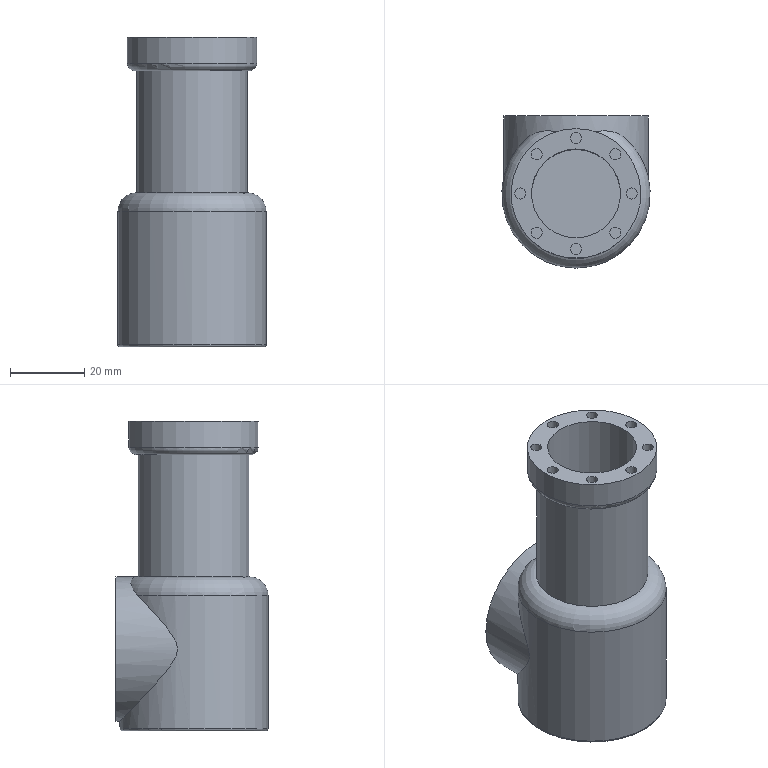Component | NX | CYLINDER | 1 solid | 32 faces | volume 51147 mm3 | cylinder 15 | plane 12 | torus 3 | cone 2 | commonest cylinder face diameters 3 x8 24 x1 40 x1 30 x1 35 x1 39 x1 3.5 x1 5 x1